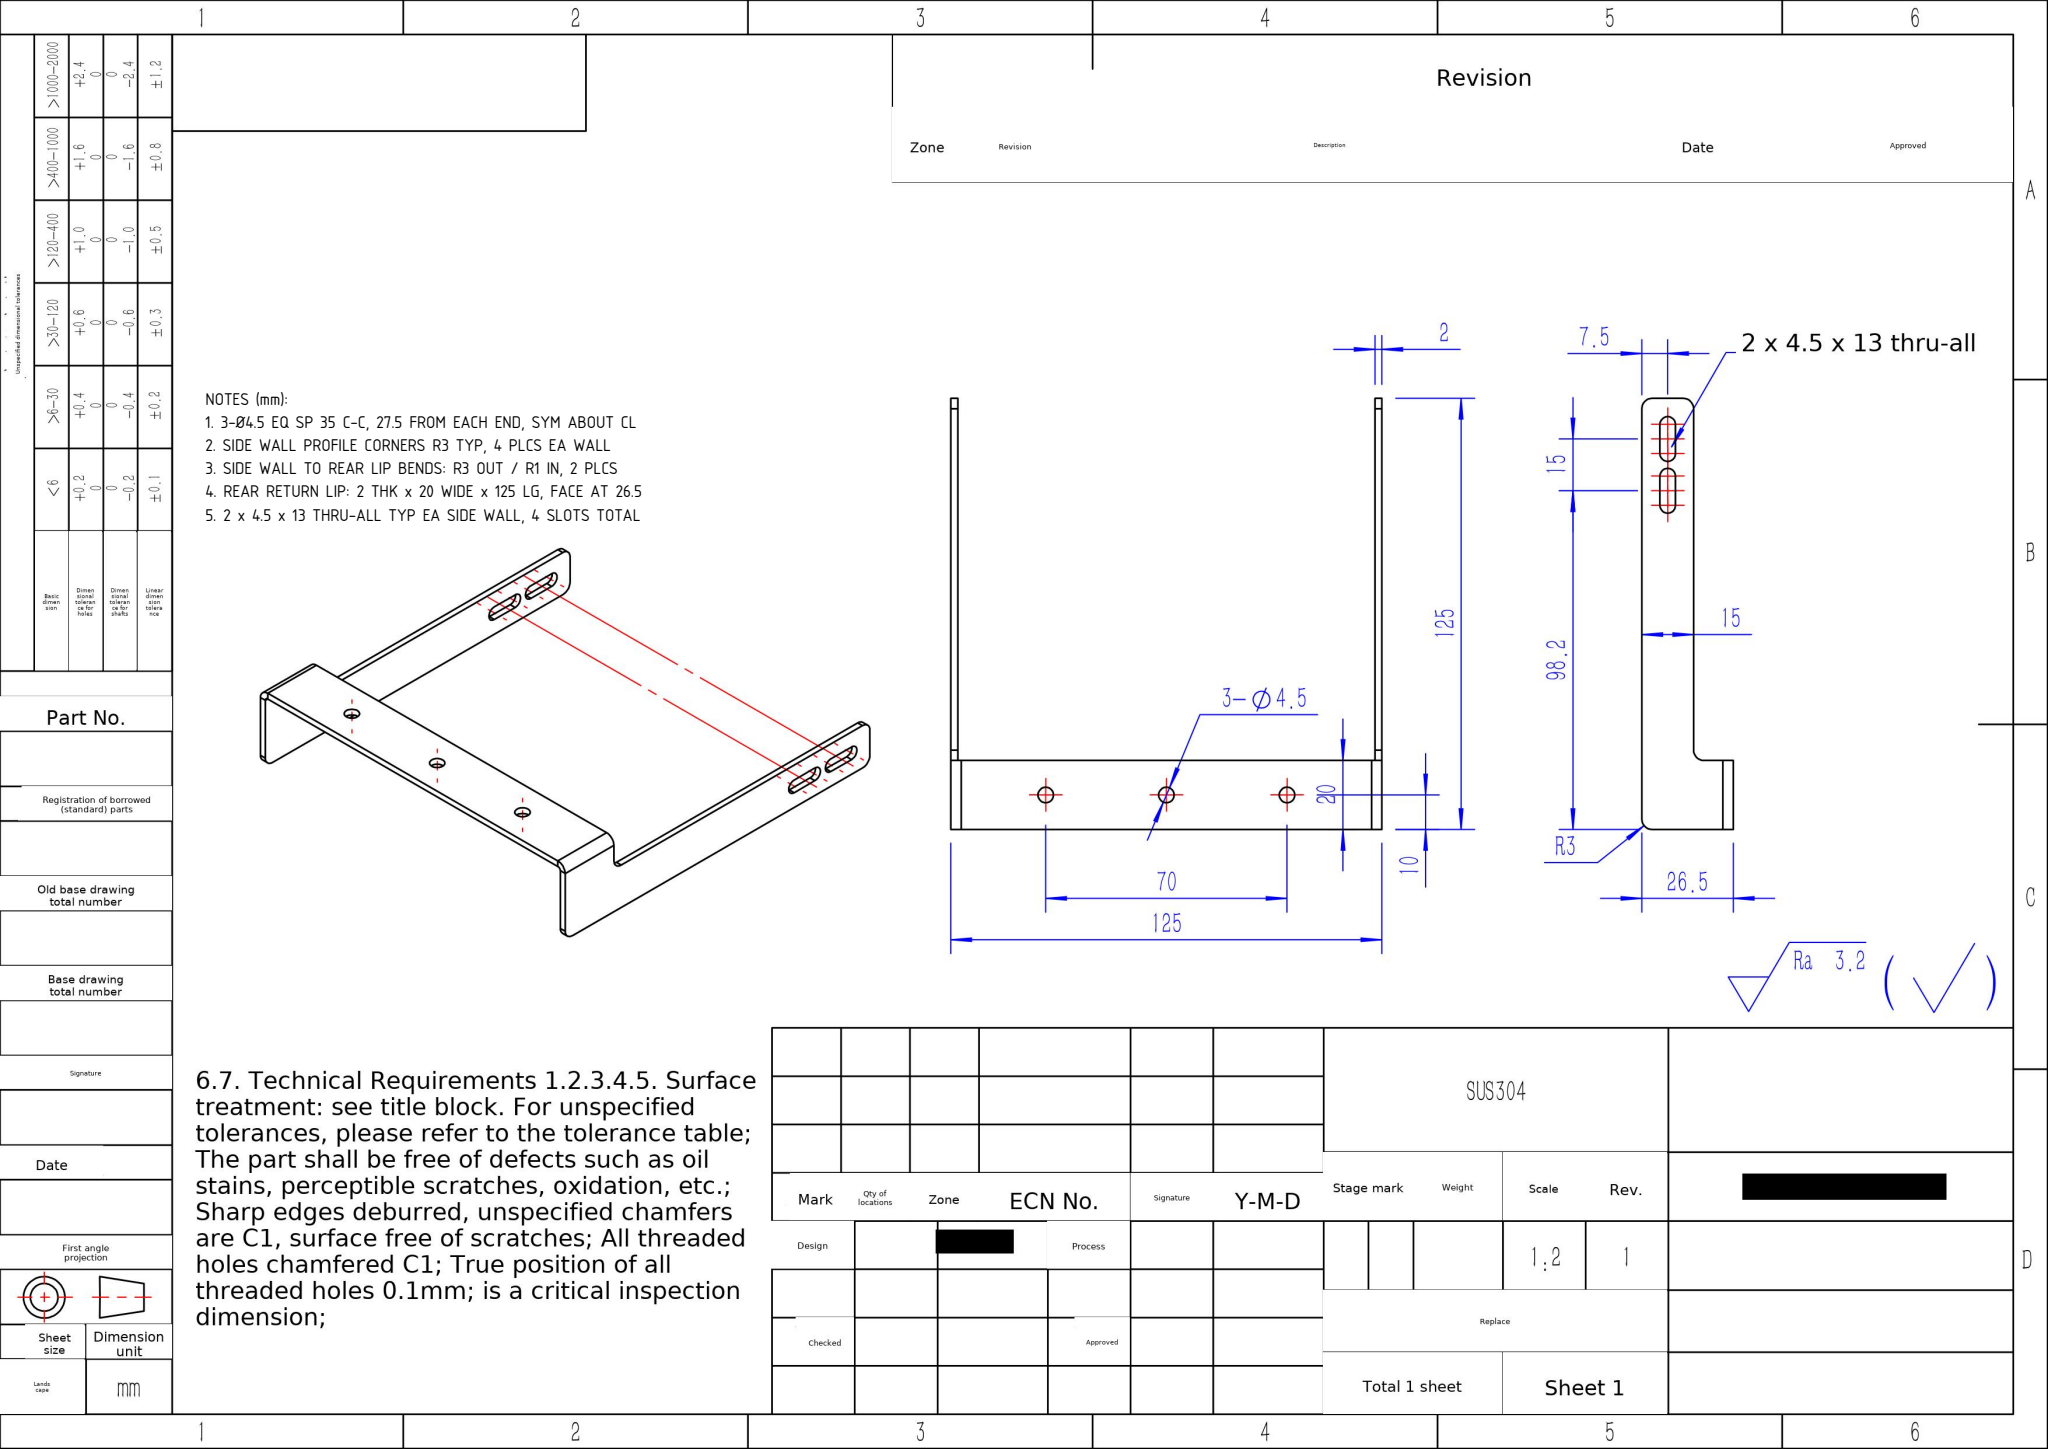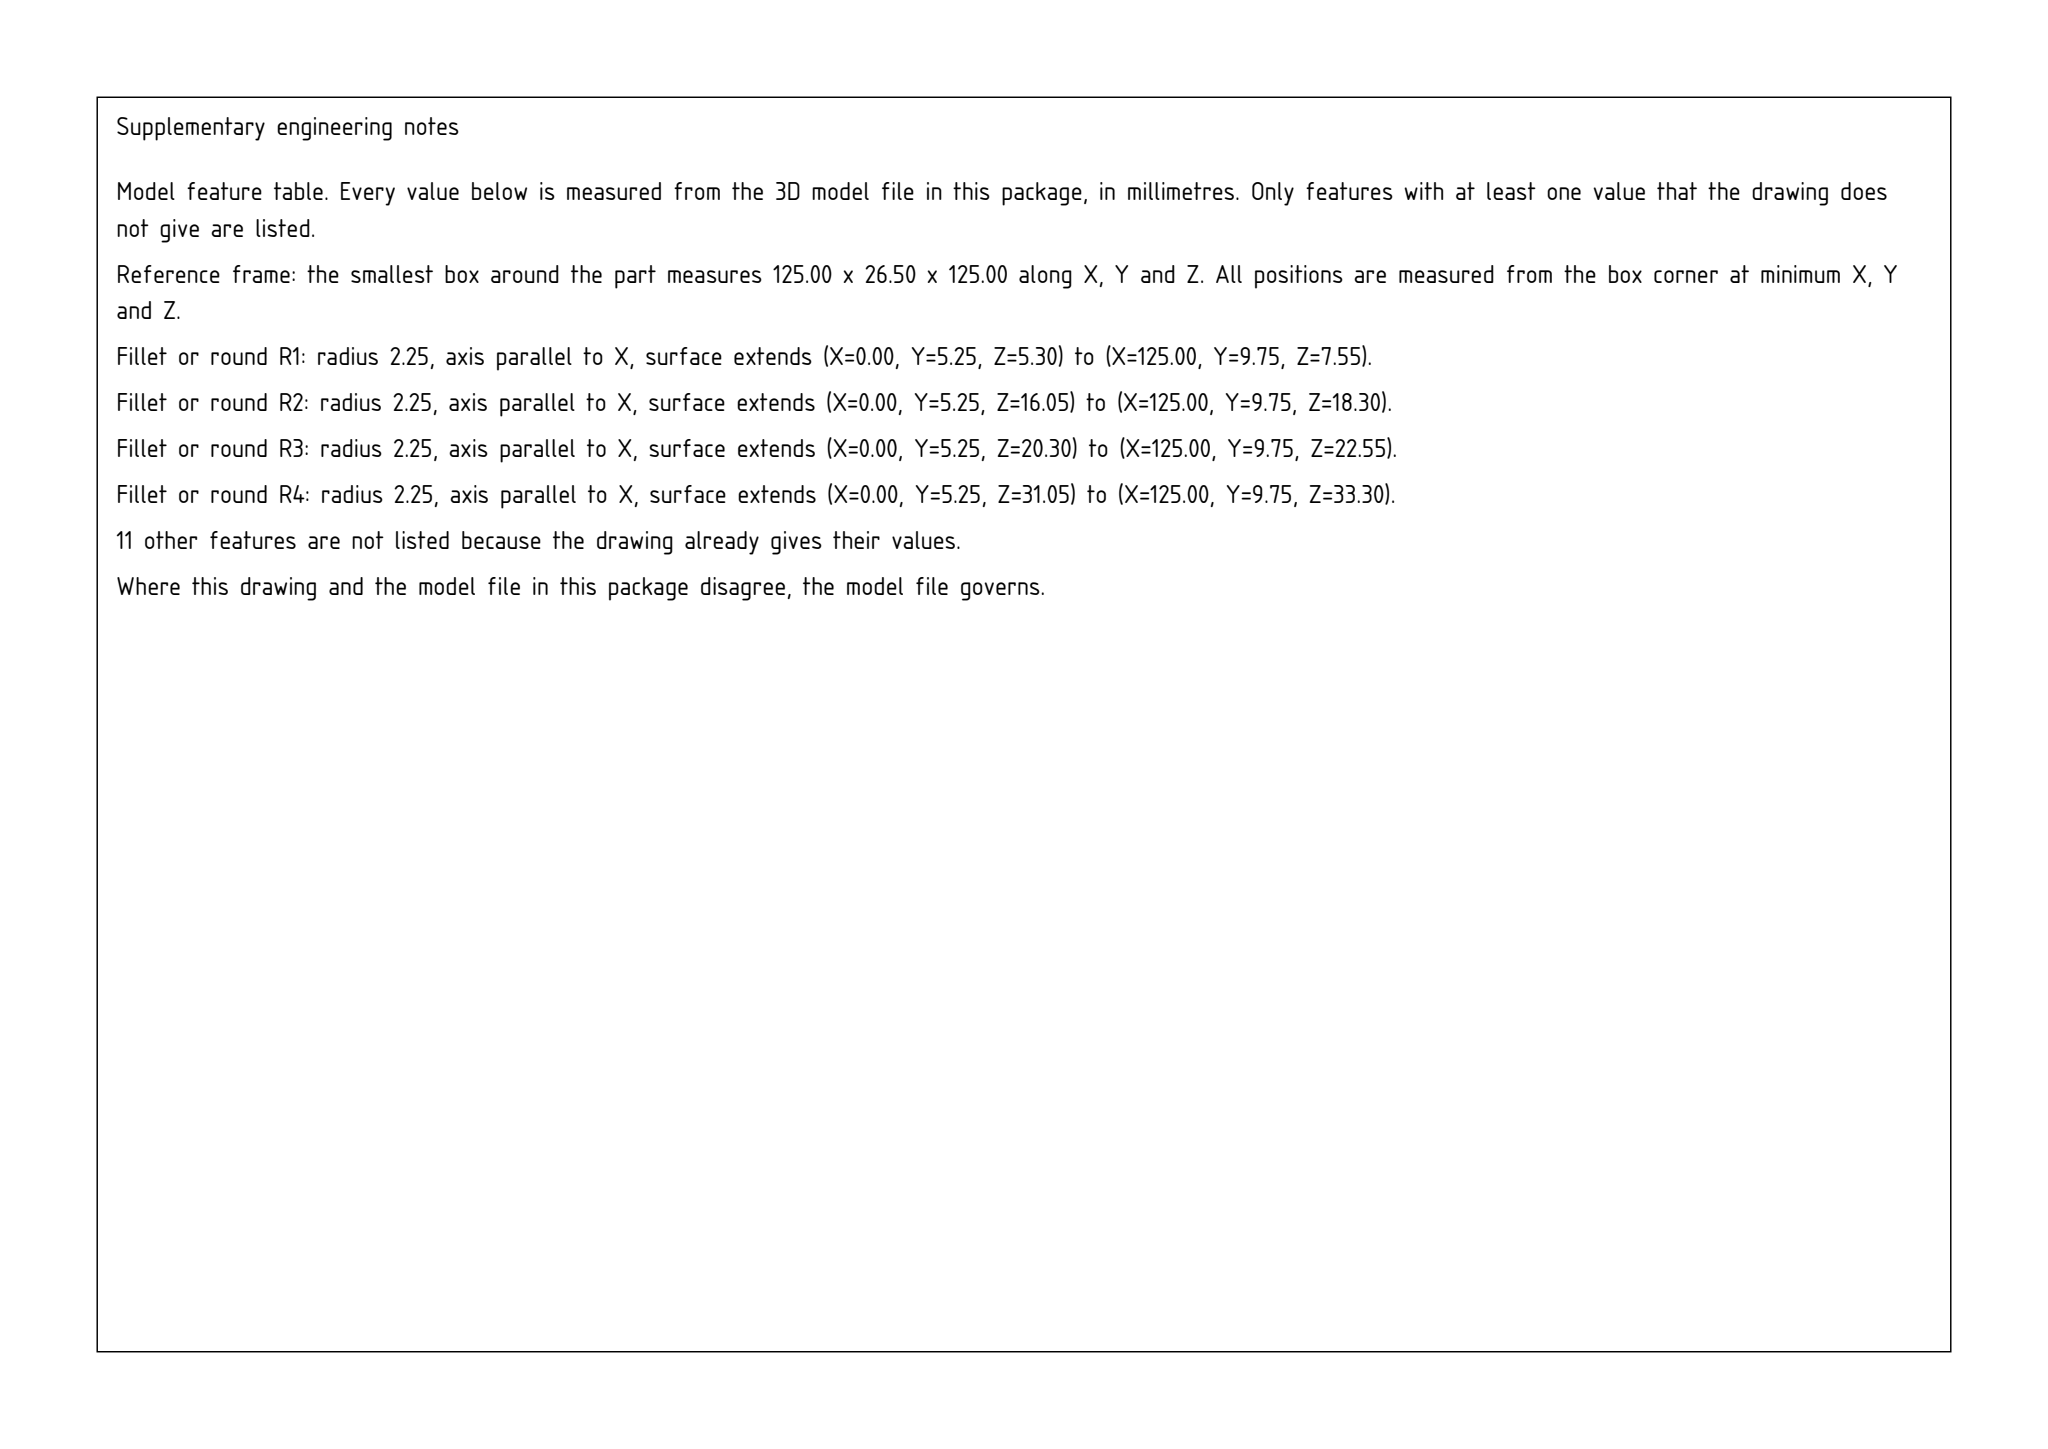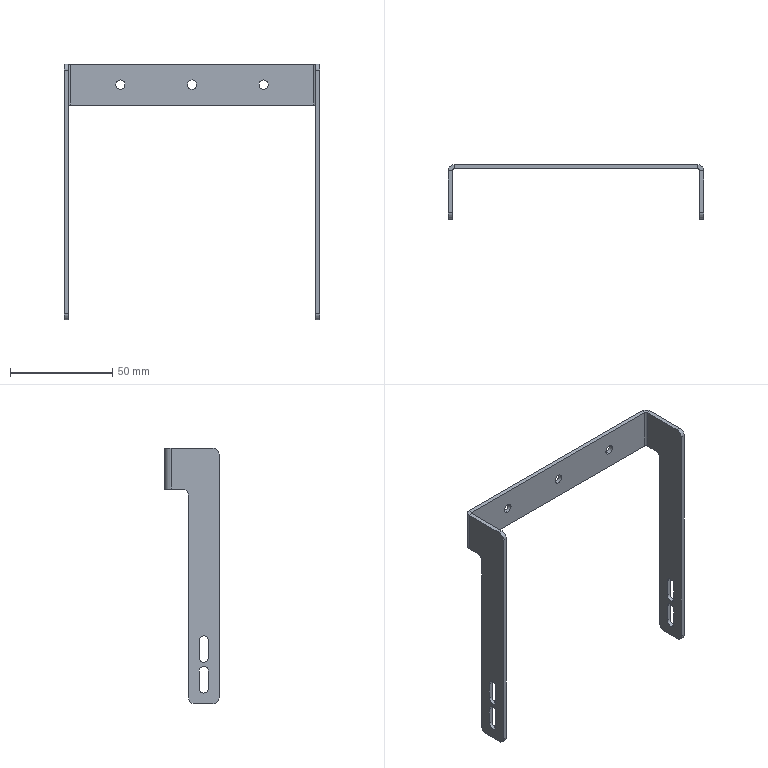Part | SolidWorks | mm | 1 solid | 60 faces | box 125 x 26.5 x 125 mm | volume 12647 mm3 | cylinder 30 | plane 30 | commonest cylinder face diameters 4.5 x18 6 x10 2 x2
Drawing notes:
3-Ø4.5 EQ SP 35 C-C, 27.5 FROM EACH END, SYM ABOUT CL | from the solid: Ø4.5 y-axis holes at z=115, x=27.5/62.5/97.5; bbox x=125; 125-97.5=27.5, spacing 35
SIDE WALL PROFILE CORNERS R3 TYP, 4 PLCS EA WALL | from the solid: 4 x Ø6.0 x-axis cyls, len 2 (=wall thk) at (y,z)=(3,3),(3,122),(12,3),(18,102), count 2 each wall
SIDE WALL TO REAR LIP BENDS: R3 OUT / R1 IN, 2 PLCS | from the solid: Ø6.0 and Ø2.0 z-axis cyls len 20 at (x,y)=(3,23.5) and (122,23.5)
REAR RETURN LIP: 2 THK x 20 WIDE x 125 LG, FACE AT 26.5 | from the solid: y planes 24.5 & 26.5, z 105-125 (20), x 0-125; bbox y=26.5
2 x 4.5 x 13 THRU-ALL TYP EA SIDE WALL, 4 SLOTS TOTAL | from the solid: Ø4.5 x-axis holes y=7.5 at z=7.55/16.05 and 22.55/31.05, mirrored at x=0-2 and x=123-125